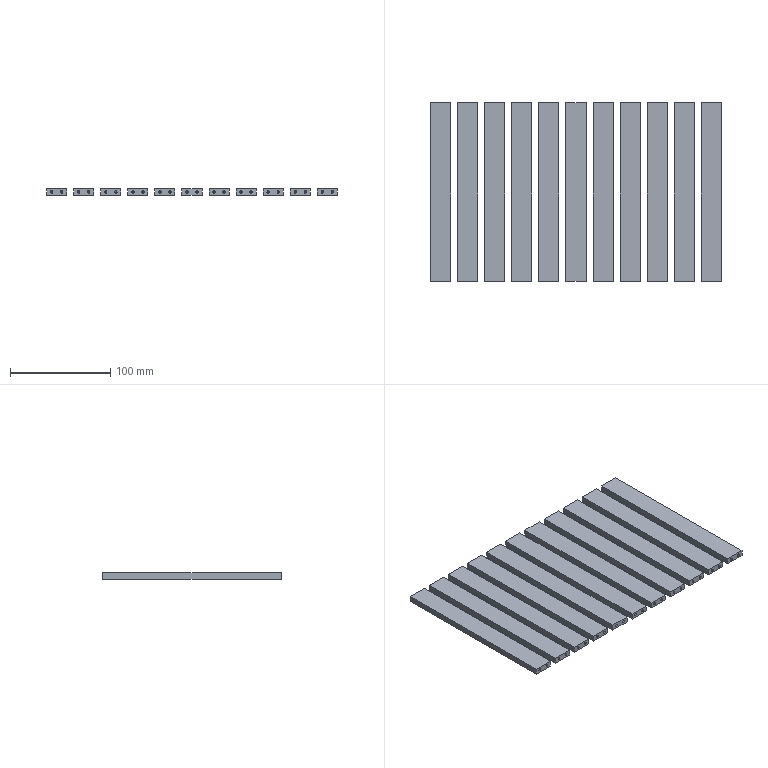CAM job | Mastercam | mm | 8 operations | part box 290 x 178 x 6
1. Contour (Ramp) | 5 - D6-C平底刀
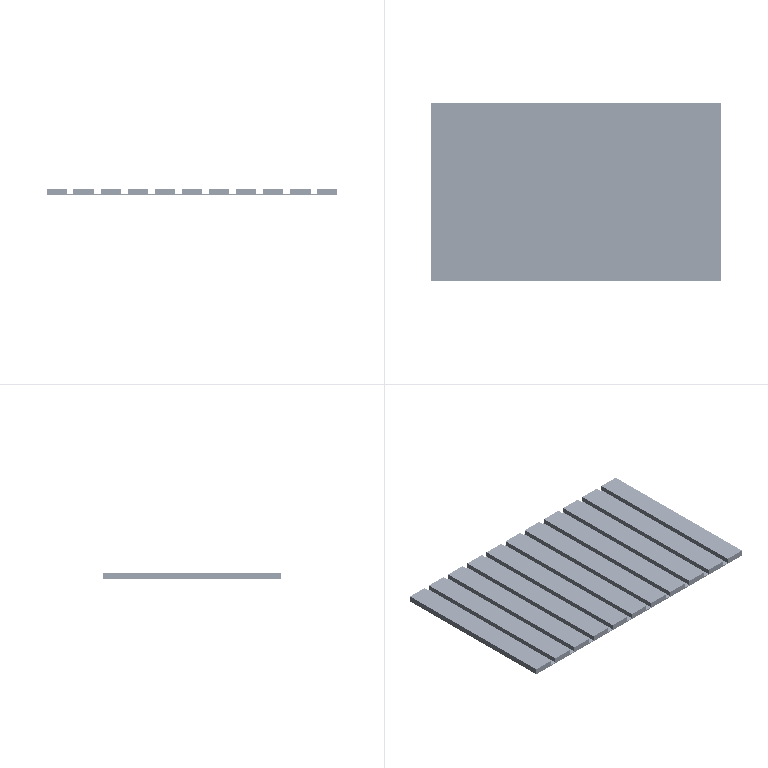2. Model Chamfer | 2 - D6定心倒角刀
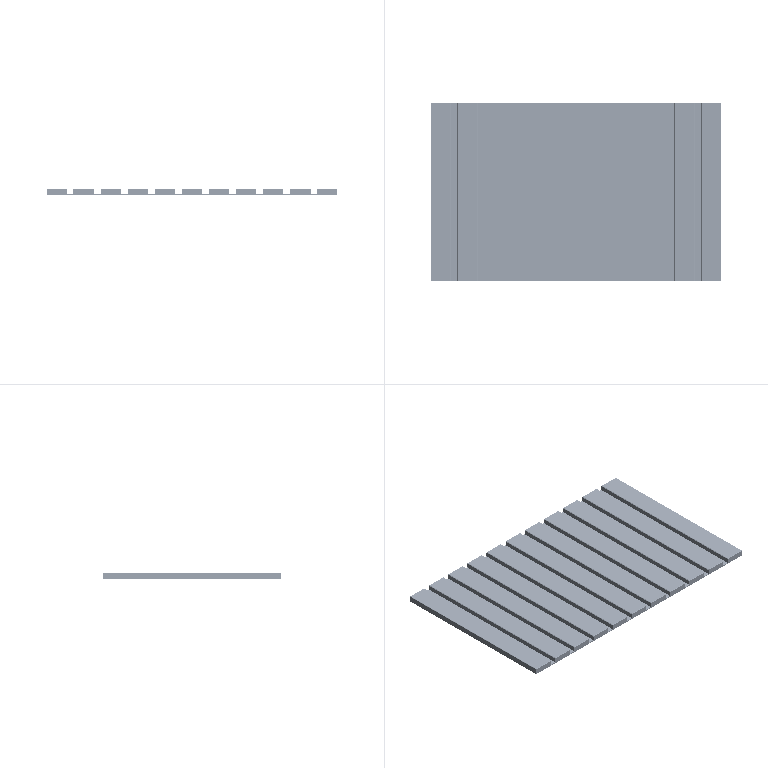3. Contour (Ramp) | 4 - D4- J平底刀
4. Model Chamfer | 2 - D6定心倒角刀
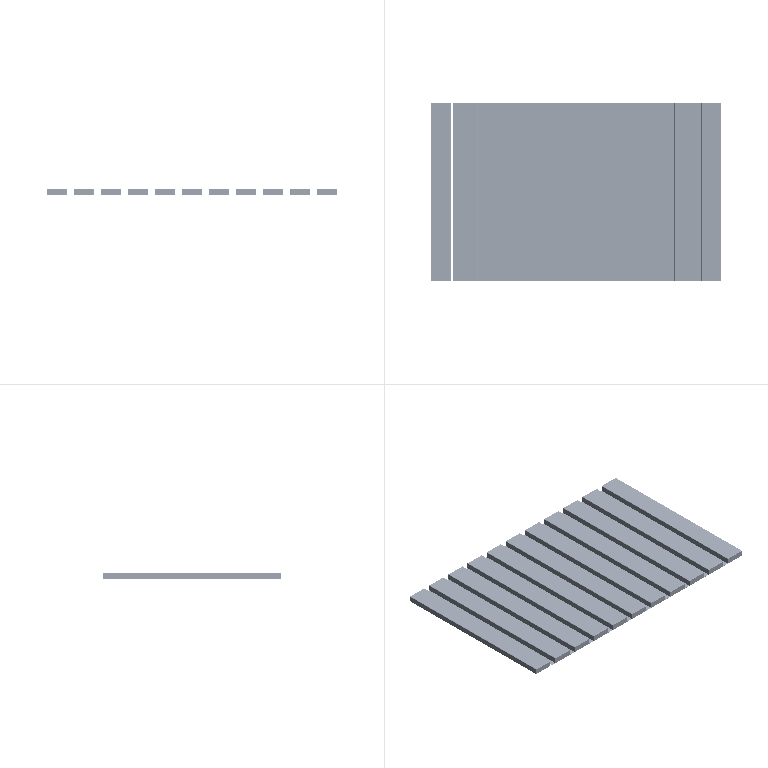5. Drill/Counterbore | 2 - D6定心倒角刀
6. Peck Drill | 16 - 2.5 钻头
7. Chamfer Drill | 2 - D6定心倒角刀
8. Thread Mill | 22 - M3/0.5  -D2.4L9螺纹铣刀